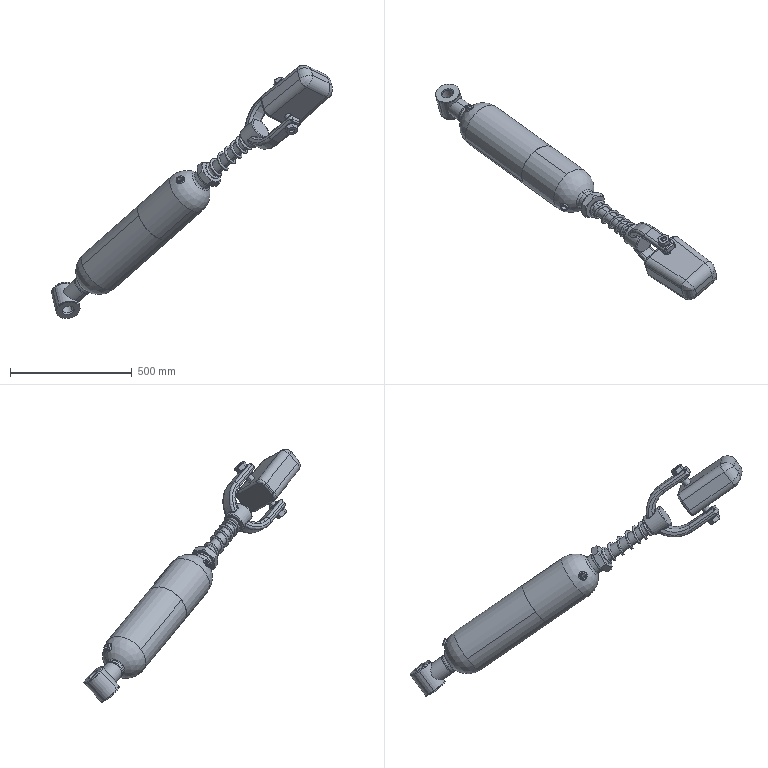Assembly | SolidWorks | mm | 22 component files | 22 solids | 495 faces | box 1153.98 x 888.42 x 1040.1 mm | volume 17215151 mm3 | cylinder 190 | plane 154 | cone 83 | spline 36 | torus 28 | sphere 4 | commonest cylinder face diameters 30 x26 20 x25 40 x24 50 x24 80 x16 60 x10 160 x10 10 x8
Bill of materials:
Bolt15x65 | 2 | Ti-3Al-8V-6Cr-4Mo-4Zr (SS) | Hexagon-headed fastener-like part with a long plain cylindrical shank and a hexagonal socket recess in the head end face.
Bolt40x20x5 | 2 | Copper | Plain flat annular washer-like disc: thin ring with a central circular through-hole.
Bolt40x60 | 1 | Ti-3Al-8V-6Cr-4Mo-4Zr (SS) | Short hexagon-headed fastener-like part with a hexagonal socket in the head and a short plain cylindrical shank.
Buffer Block^LandingGearAssembly | 1 |  | Rectangular block with heavily rounded edges and corners and a small round hole.
BufferSpring2 | 1 | Chrome Stainless Steel | Helical coil spring-like part made of round wire with open, unground ends, about 8 turns.
ConnectingPlate | 1 | Copper | Thick circular disc with concentric half-circle arc steps or ribs on one face and a small short cylindrical stub near the center.
Connector | 1 | Ti-3Al-8V-6Cr-4Mo-4Zr (SS) | Two intersecting hollow cylindrical tube sections joined at an angle, like a branched or elbow-type fitting body, each with a bore.
DampingSpring | 1 | Chrome Stainless Steel | Helical coil spring-like part made of round wire with open ends, about 6 turns and fairly open pitch.
FlatWasher15x50x2.5 | 4 | Copper | Stepped annular washer: two stacked thin rings with different outer diameters sharing a common central through-hole.
FrictionWasher | 1 | Copper | Thick cylindrical spool- or bushing-like body with a central bore and two shallow circumferential grooves on the outer surface.
FrictionWasher2 | 2 | Copper | Stepped annular washer: a thin ring with a thinner, smaller-diameter ring step on one face and a common central through-hole.
Gasket | 1 | Copper | Thin-walled cylindrical ring or short sleeve with a large bore and short axial length.
Gasket2 | 1 | Ti-3Al-8V-6Cr-4Mo-4Zr (SS) | Hexagonal prism with a plain cylindrical through-bore and a short cylindrical collar or boss on one face. It is shaped like a hex nut with a collar.
Sleeve | 1 | 201.0-T7 Insulated Mold Casting (SS) | Thin-walled cylindrical shell with a domed closed end and a fully open opposite end. The dome carries a small central boss with a hole and a second small offset boss with a hole.
SpringSleeve | 1 | 201.0-T7 Insulated Mold Casting (SS) | Closed cylindrical vessel-like body with a domed end. The dome has a central short tubular neck and a small offset boss with a hole. A slight step in diameter appears along the cylindrical body.
Strut | 1 | 201.0-T7 Insulated Mold Casting (SS) | Long slender cylindrical rod with a curved U-shaped fork (yoke) at one end. A cylindrical hub joins the rod to the fork, and each fork arm ends in a flat tab with a through-hole.
Mates:
1. coincident | FlatWasher15x50x2.5-6 face at (523.806, -2110.295, 812.667) dir (-0.1878, 0.645, 0.7408) | Strut-1 face at (483.024, -2047.115, 747.321) dir (0.1878, -0.645, -0.7408)
2. concentric | Strut-1 face at (555.733, -2219.937, 686.733) dir (0.1878, -0.645, -0.7408) r 15 | FlatWasher15x50x2.5-7 face at (560.898, -2237.673, 666.361) dir (0.1878, -0.645, -0.7408) r 15
3. coincident | Strut-1 face at (560.898, -2237.673, 666.361) dir (0.1878, -0.645, -0.7408) | FlatWasher15x50x2.5-7 face at (560.898, -2237.673, 666.361) dir (-0.1878, 0.645, 0.7408)
4. concentric | Strut-1 face at (523.806, -2110.295, 812.667) dir (-0.1878, 0.645, 0.7408) r 15 | FlatWasher15x50x2.5-8 face at (518.642, -2092.559, 833.038) dir (-0.1878, 0.645, 0.7408) r 15
5. coincident | Strut-1 face at (518.642, -2092.559, 833.038) dir (-0.1878, 0.645, 0.7408) | FlatWasher15x50x2.5-8 face at (518.642, -2092.559, 833.038) dir (0.1878, -0.645, -0.7408)
6. concentric | Strut-1 face at (555.733, -2219.937, 686.733) dir (0.1878, -0.645, -0.7408) r 15 | Bolt15x65-1 face at (543.995, -2179.627, 733.032) dir (0.1878, -0.645, -0.7408) r 15
7. coincident | FlatWasher15x50x2.5-7 face at (561.837, -2240.898, 662.657) dir (0.1878, -0.645, -0.7408) | Bolt15x65-1 face at (561.837, -2240.898, 662.657) dir (-0.1878, 0.645, 0.7408)
8. concentric | Strut-1 face at (523.806, -2110.295, 812.667) dir (-0.1878, 0.645, 0.7408) r 15 | Bolt15x65-2 face at (535.544, -2150.605, 766.368) dir (-0.1878, 0.645, 0.7408) r 15
9. coincident | FlatWasher15x50x2.5-8 face at (517.703, -2089.334, 836.742) dir (-0.1878, 0.645, 0.7408) | Bolt15x65-2 face at (517.703, -2089.334, 836.742) dir (0.1878, -0.645, -0.7408)
10. concentric | Strut-1 face at (-71.787, -1723.224, 209.935) dir (0.6592, -0.4763, 0.5818) r 25 | SpringSleeve-1 face at (163.816, -1893.464, 417.88) dir (0.6592, -0.4763, 0.5818) r 25
11. concentric | SpringSleeve-1 face at (-63.616, -1729.129, 217.147) dir (0.6592, -0.4763, 0.5818) r 87.5 | Sleeve-1 face at (2.307, -1776.762, 275.33) dir (-0.6592, 0.4763, -0.5818) r 87.5
12. coincident | SpringSleeve-1 face at (2.307, -1776.762, 275.33) dir (-0.6592, 0.4763, -0.5818) | Sleeve-1 face at (2.307, -1776.762, 275.33) dir (0.6592, -0.4763, 0.5818)
13. concentric | Strut-1 face at (-71.787, -1723.224, 209.935) dir (0.6592, -0.4763, 0.5818) r 25 | Gasket-1 face at (188.537, -1911.326, 439.699) dir (0.6592, -0.4763, 0.5818) r 25
14. coincident | SpringSleeve-1 face at (188.537, -1911.326, 439.699) dir (0.6592, -0.4763, 0.5818) | Gasket-1 face at (188.537, -1911.326, 439.699) dir (-0.6592, 0.4763, -0.5818)
15. concentric | Strut-1 face at (-71.787, -1723.224, 209.935) dir (0.6592, -0.4763, 0.5818) r 25 | Gasket2-1 face at (195.459, -1916.328, 445.808) dir (0.6592, -0.4763, 0.5818) r 25
16. coincident | Gasket-1 face at (195.459, -1916.328, 445.808) dir (0.6592, -0.4763, 0.5818) | Gasket2-1 face at (195.459, -1916.328, 445.808) dir (-0.6592, 0.4763, -0.5818)
17. concentric | Strut-1 face at (-71.787, -1723.224, 209.935) dir (0.6592, -0.4763, 0.5818) r 25 | FrictionWasher-1 face at (-48.714, -1739.896, 230.299) dir (-0.6592, 0.4763, -0.5818) r 25
18. coincident | Strut-1 face at (-71.787, -1723.224, 209.935) dir (-0.6592, 0.4763, -0.5818) | FrictionWasher-1 face at (-71.787, -1723.224, 209.935) dir (0.6592, -0.4763, 0.5818)
19. concentric | Strut-1 face at (-71.787, -1723.224, 209.935) dir (0.6592, -0.4763, 0.5818) r 25 | BufferSpring2-1 sketch segment at (381.956, -2051.085, 610.412) dir (-0.6592, 0.4763, -0.5818) r 32.5
20. coincident | Strut-1 face at (384.106, -2052.937, 613.334) dir (-0.6592, 0.4763, -0.5818) | BufferSpring2-1 face at (384.593, -2052.99, 612.739) dir (0.6592, -0.4763, 0.5818)
21. concentric | Sleeve-1 face at (-277.863, -1574.32, 28.05) dir (-0.6592, 0.4763, -0.5818) r 20 | Bolt40x60-1 face at (-327.305, -1538.595, -15.587) dir (0.6592, -0.4763, 0.5818) r 20
22. concentric | Bolt40x60-1 face at (-327.305, -1538.595, -15.587) dir (0.6592, -0.4763, 0.5818) r 20 | Bolt40x20x5-1 face at (-297.64, -1560.03, 10.595) dir (0.6592, -0.4763, 0.5818) r 20
23. concentric | Bolt40x60-1 face at (-327.305, -1538.595, -15.587) dir (0.6592, -0.4763, 0.5818) r 20 | Bolt40x20x5-2 face at (-274.567, -1576.702, 30.96) dir (0.6592, -0.4763, 0.5818) r 20
24. coincident | Bolt40x60-1 face at (-271.271, -1579.084, 33.869) dir (-0.6592, 0.4763, -0.5818) | Bolt40x20x5-2 face at (-271.271, -1579.084, 33.869) dir (0.6592, -0.4763, 0.5818)
25. coincident | Sleeve-1 face at (-294.344, -1562.412, 13.505) dir (-0.6592, 0.4763, -0.5818) | Bolt40x20x5-1 face at (-294.344, -1562.412, 13.505) dir (0.6592, -0.4763, 0.5818)
26. concentric | Bolt40x60-1 face at (-327.305, -1538.595, -15.587) dir (0.6592, -0.4763, 0.5818) r 20 | Connector-1 face at (-340.489, -1529.069, -27.224) dir (0.6592, -0.4763, 0.5818) r 20
27. coincident | Bolt40x20x5-1 face at (-297.64, -1560.03, 10.595) dir (-0.6592, 0.4763, -0.5818) | Connector-1 face at (-297.64, -1560.03, 10.595) dir (0.6592, -0.4763, 0.5818)
28. coincident | Bolt40x60-1 edge at (-327.305, -1538.595, -15.587) dir (-0.6592, 0.4763, -0.5818) r 20 | ConnectingPlate-1 face at (-330.601, -1536.214, -18.496) dir (0.6592, -0.4763, 0.5818) r 20
29. coincident | Bolt40x60-1 face at (-327.305, -1538.595, -15.587) dir (-0.6592, 0.4763, -0.5818) | ConnectingPlate-1 face at (-327.305, -1538.595, -15.587) dir (0.6592, -0.4763, 0.5818)
30. concentric | Connector-1 face at (-372.314, -1479.632, -10.848) dir (0.175, -0.6553, -0.7348) r 25 | FrictionWasher2-2 face at (-371.439, -1482.908, -14.522) dir (-0.175, 0.6553, 0.7348) r 25
31. coincident | Connector-1 face at (-371.439, -1482.908, -14.522) dir (-0.175, 0.6553, 0.7348) | FrictionWasher2-2 face at (-371.439, -1482.908, -14.522) dir (0.175, -0.6553, -0.7348)
32. concentric | Connector-1 face at (-372.314, -1479.632, -10.848) dir (0.175, -0.6553, -0.7348) r 25 | FrictionWasher2-1 face at (-355.685, -1541.886, -80.654) dir (0.175, -0.6553, -0.7348) r 25
33. coincident | Connector-1 face at (-355.685, -1541.886, -80.654) dir (0.175, -0.6553, -0.7348) | FrictionWasher2-1 face at (-355.685, -1541.886, -80.654) dir (-0.175, 0.6553, 0.7348)
34. coincident | SpringSleeve-1 face at (173.704, -1900.609, 426.607) dir (-0.6592, 0.4763, -0.5818) | DampingSpring-2 face at (173.704, -1900.609, 426.607) dir (0.6592, -0.4763, 0.5818)
35. concentric | Strut-1 face at (-71.787, -1723.224, 209.935) dir (0.6592, -0.4763, 0.5818) r 25 | DampingSpring-2 sketch segment at (171.067, -1898.703, 424.28) dir (-0.6592, 0.4763, -0.5818) r 32.5
36. distance | FrictionWasher-1 face at (-48.714, -1739.896, 230.299) dir (0.6592, -0.4763, 0.5818) | DampingSpring-2 face at (72.184, -1827.253, 337.005) dir (-0.6592, 0.4763, -0.5818)
37. concentric | FlatWasher15x50x2.5-6 face at (524.745, -2113.52, 808.963) dir (-0.1878, 0.645, 0.7408) r 15 | Bolt15x65-2 face at (535.544, -2150.605, 766.368) dir (-0.1878, 0.645, 0.7408) r 15
38. concentric | FlatWasher15x50x2.5-5 face at (554.794, -2216.712, 690.437) dir (0.1878, -0.645, -0.7408) r 15 | Bolt15x65-1 face at (543.995, -2179.627, 733.032) dir (0.1878, -0.645, -0.7408) r 15
39. coincident | FlatWasher15x50x2.5-5 face at (555.733, -2219.937, 686.733) dir (0.1878, -0.645, -0.7408) | Strut-1 face at (514.951, -2156.757, 621.387) dir (-0.1878, 0.645, 0.7408)
40. distance | BufferSpring2-1 face at (233.631, -1943.91, 479.499) dir (-0.6592, 0.4763, -0.5818) | Gasket2-1 face at (233.364, -1943.717, 479.264) dir (0.6592, -0.4763, 0.5818)
41. concentric | Bolt15x65-1 face at (543.995, -2179.627, 733.032) dir (0.1878, -0.645, -0.7408) r 15 | Buffer Block^LandingGearAssembly-1 face at (529.441, -2129.644, 790.443) dir (0.1878, -0.645, -0.7408) r 15
42. width | Buffer Block^LandingGearAssembly-1 face at (696.145, -4884.068, 3082.294) dir (0.1878, -0.645, -0.7408) | Buffer Block^LandingGearAssembly-1 face at (675.486, -4813.123, 3163.781) dir (-0.1878, 0.645, 0.7408) | Strut-1 face at (474.094, -2025.385, 766.636) dir (-0.1878, 0.645, 0.7408) | Strut-1 face at (517.289, -2173.724, 596.254) dir (0.1878, -0.645, -0.7408)
43. coincident | Sleeve-1 face at (-274.567, -1576.702, 30.96) dir (0.6592, -0.4763, 0.5818) | Bolt40x20x5-2 face at (-274.567, -1576.702, 30.96) dir (-0.6592, 0.4763, -0.5818)